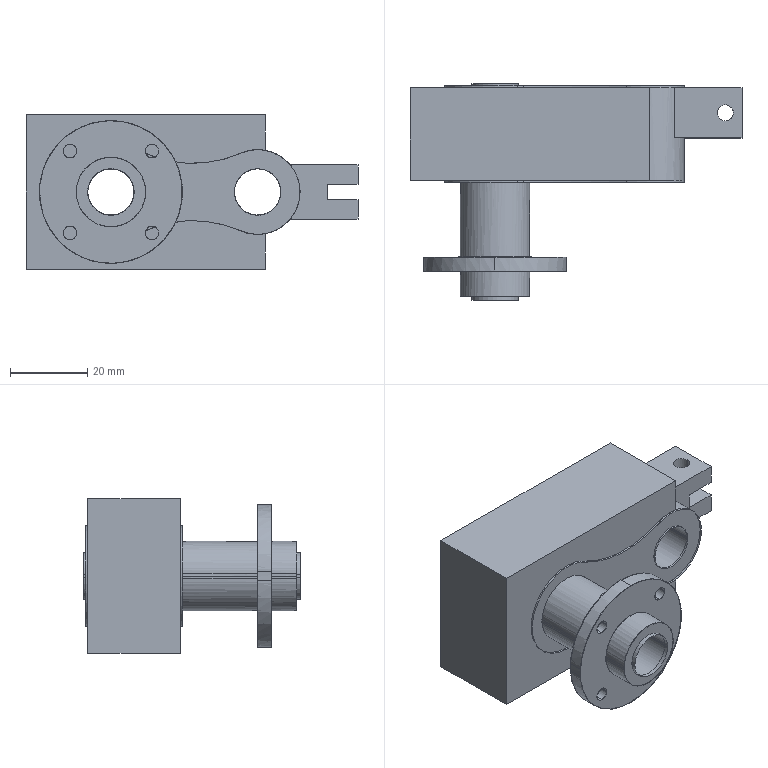CAM job | Mastercam | mm | 14 operations | part box 86 x 56.16 x 40
1. Facing | 24 - 100 平底刀
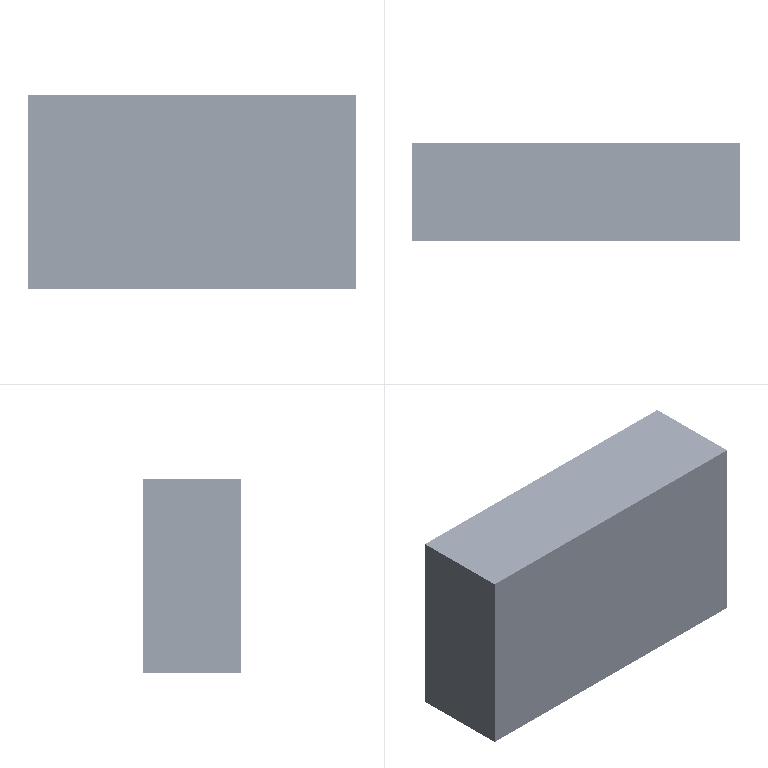2. 2D High Speed (2D Dynamic Mill) | 10 - 10 平底刀
3. Contour (Ramp) | 10 - 10 平底刀
4. Contour (2D) | 10 - 10 平底刀
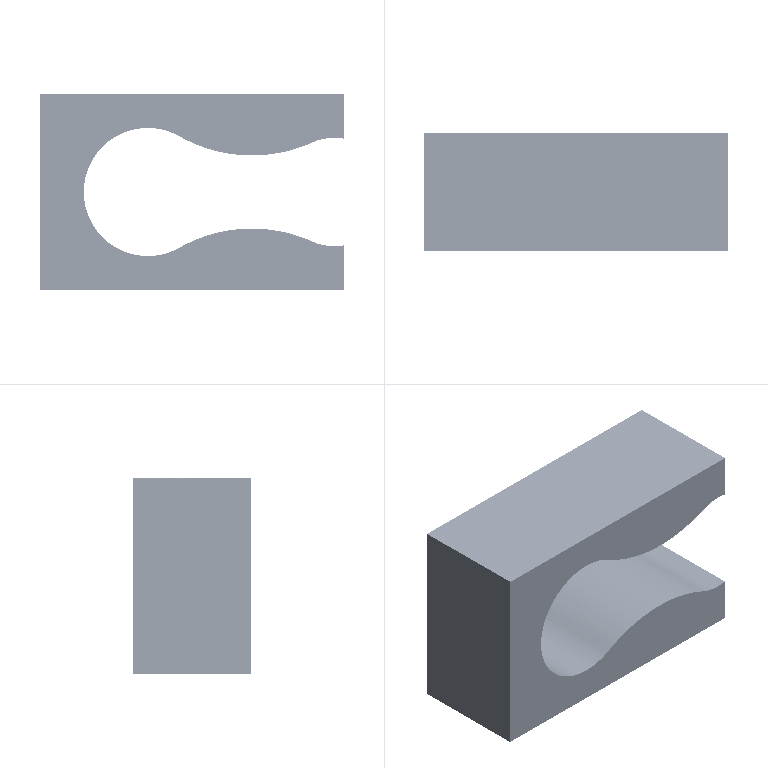5. Contour (2D chamfer) | 7 - 6 倒角刀
6. Facing | 24 - 100 平底刀
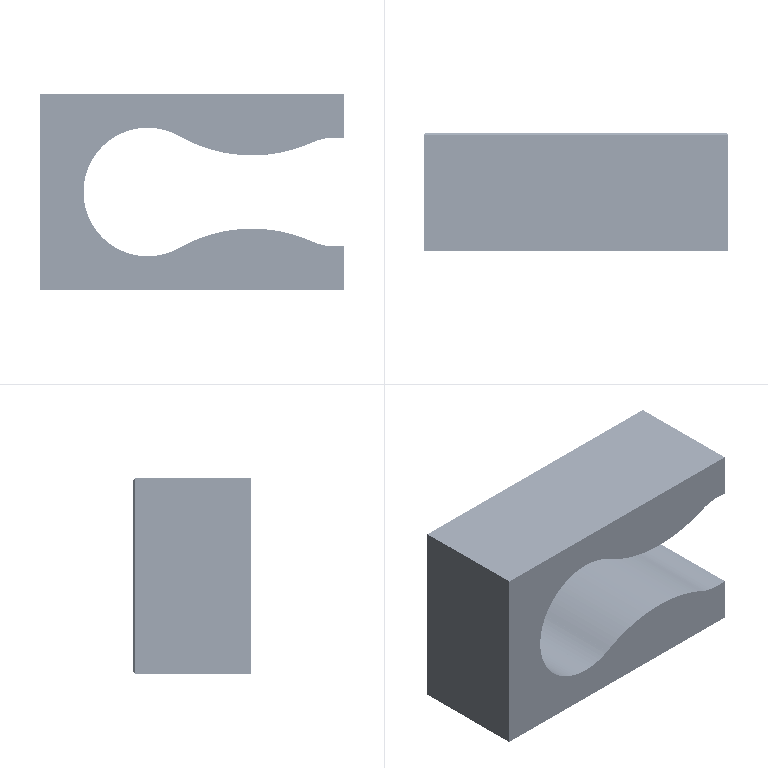7. Facing | 24 - 100 平底刀
8. Drill/Counterbore | 7 - 6 倒角刀
9. Peck Drill | 1 - 4.2 钻头
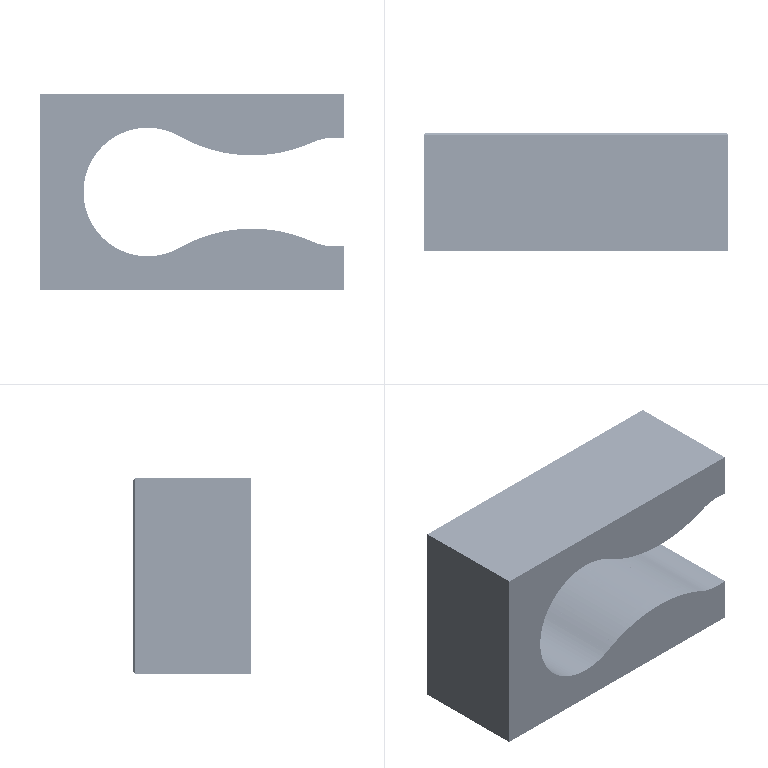10. Contour (Ramp) | 3 - 3 平底刀
11. Contour (2D) | 3 - 3 平底刀
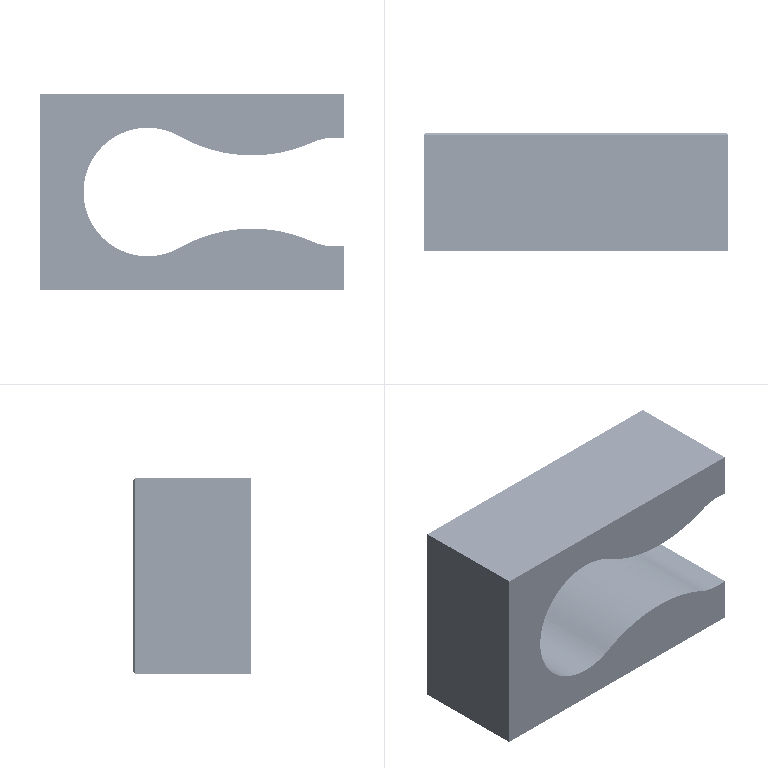12. Contour (Ramp) | 3 - 3 平底刀
13. Contour (Ramp) | 3 - 3 平底刀
14. Contour (2D chamfer) | 7 - 6 倒角刀